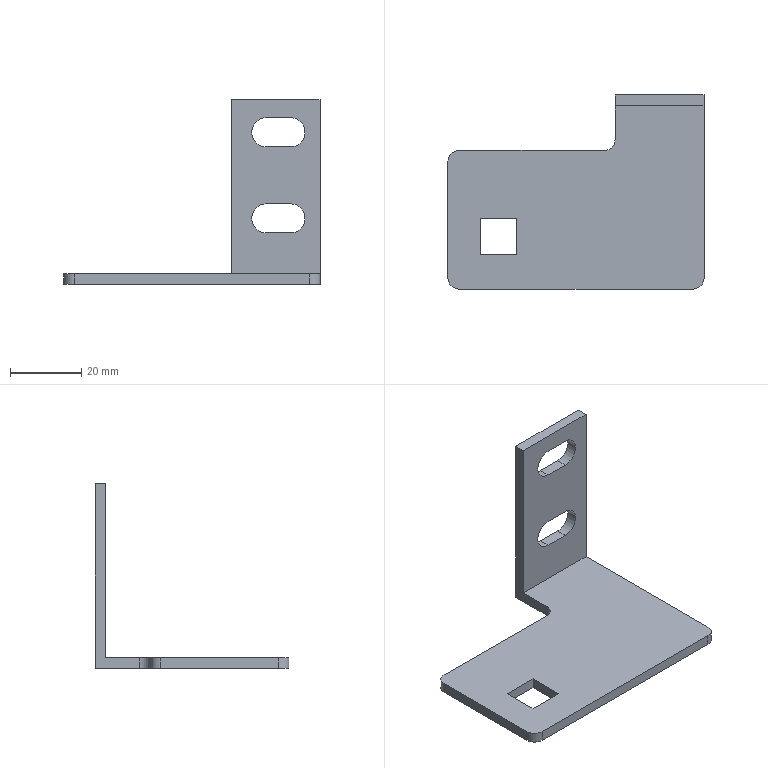Component | SolidWorks | MotorHeadBracket-1 | 1 solid | 26 faces | box 72 x 54.5 x 52 mm | volume 12286 mm3 | plane 18 | cylinder 8 | commonest cylinder face diameters 6 x4 8.2 x4
build123d program:
from build123d import *

# Parameters (mm, degrees)
SKETCH2_W           = 10.2
SKETCH2_H           = 10.2
BOSS_EXTRUDE1_DEPTH = 3
FILLET1_R           = 3
SKETCH3_W           = 25
SKETCH3_H           = 3
BOSS_EXTRUDE2_DEPTH = 52
CUT_EXTRUDE1_DEPTH  = 12


with BuildPart() as part:
    # Sketch2 → Boss-Extrude1 (new body)
    with BuildSketch(Plane.XY):
        Polygon((0, 0), (0, 39), (47, 39), (47, 54.5), (72, 54.5), (72, 0), align=None)
        with Locations((14.2, 14.8)):
            Rectangle(SKETCH2_W, SKETCH2_H, mode=Mode.SUBTRACT)
    extrude(amount=BOSS_EXTRUDE1_DEPTH)

    # Fillet1
    fillet1_edges = [part.edges().sort_by_distance(p)[0] for p in [
        (0, 0, 1.5),
        (0, 39, 1.5),
        (47, 39, 1.5),
        (72, 0, 1.5),
    ]]
    fillet(fillet1_edges, radius=FILLET1_R)

    # Sketch3 → Boss-Extrude2 (add)
    with BuildSketch(Plane.XY):
        with Locations((59.5, 53)):
            Rectangle(SKETCH3_W, SKETCH3_H)
    extrude(amount=BOSS_EXTRUDE2_DEPTH)

    # Sketch4 → Cut-Extrude1 (cut)
    with BuildSketch(Plane(origin=(0, 54.5, 0), x_dir=(1, 0, 0), z_dir=(0, 1, 0))):
        with BuildLine():
            Line((63.7, -46.9), (56.9, -46.9))
            ThreePointArc((56.9, -46.9), (52.8, -42.8), (56.9, -38.7))
            Line((56.9, -38.7), (63.7, -38.7))
            ThreePointArc((63.7, -38.7), (67.8, -42.8), (63.7, -46.9))
        make_face()
        with BuildLine():
            Line((63.7, -22.7), (56.9, -22.7))
            ThreePointArc((56.9, -22.7), (52.8, -18.6), (56.9, -14.5))
            Line((56.9, -14.5), (63.7, -14.5))
            ThreePointArc((63.7, -14.5), (67.8, -18.6), (63.7, -22.7))
        make_face()
    extrude(amount=-CUT_EXTRUDE1_DEPTH, mode=Mode.SUBTRACT)


solid = part.part

# Placed as in the assembly
solid = solid.moved(Location((-79.293, -47.753, 1574.064), (0, 0, 0)))
STEP:
#1=COLOUR_RGB('',0.7922,0.8196,0.9333);
#2=FILL_AREA_STYLE_COLOUR('',#1);
#3=FILL_AREA_STYLE('',(#2));
#4=SURFACE_STYLE_FILL_AREA(#3);
#5=SURFACE_SIDE_STYLE('',(#4));
#6=SURFACE_STYLE_USAGE(.BOTH.,#5);
#7=PRESENTATION_STYLE_ASSIGNMENT((#6));
#8=CARTESIAN_POINT('',(-2.362,-1.498,62.089));
#9=VERTEX_POINT('',#8);
#10=CARTESIAN_POINT('',(-2.362,-1.097,62.089));
#11=VERTEX_POINT('',#10);
#12=CARTESIAN_POINT('',(-2.362,-1.097,62.089));
#13=DIRECTION('',(0.,1.,0.));
#14=VECTOR('',#13,39.37);
#15=LINE('',#12,#14);
#16=EDGE_CURVE('',#9,#11,#15,.T.);
#17=ORIENTED_EDGE('',*,*,#16,.F.);
#18=CARTESIAN_POINT('',(-2.764,-1.498,62.089));
#19=VERTEX_POINT('',#18);
#20=CARTESIAN_POINT('',(-2.764,-1.498,62.089));
#21=DIRECTION('',(1.,0.,0.));
#22=VECTOR('',#21,39.37);
#23=LINE('',#20,#22);
#24=EDGE_CURVE('',#19,#9,#23,.T.);
#25=ORIENTED_EDGE('',*,*,#24,.F.);
#26=CARTESIAN_POINT('',(-2.764,-1.097,62.089));
#27=VERTEX_POINT('',#26);
#28=CARTESIAN_POINT('',(-2.764,-1.097,62.089));
#29=DIRECTION('',(0.,-1.,0.));
#30=VECTOR('',#29,39.37);
#31=LINE('',#28,#30);
#32=EDGE_CURVE('',#27,#19,#31,.T.);
#33=ORIENTED_EDGE('',*,*,#32,.F.);
#34=CARTESIAN_POINT('',(-2.764,-1.097,62.089));
#35=DIRECTION('',(-1.,-0.,0.));
#36=VECTOR('',#35,39.37);
#37=LINE('',#34,#36);
#38=EDGE_CURVE('',#11,#27,#37,.T.);
#39=ORIENTED_EDGE('',*,*,#38,.F.);
#40=EDGE_LOOP('',(#17,#25,#33,#39));
#41=FACE_BOUND('',#40,.T.);
#42=CARTESIAN_POINT('',(-1.271,0.1475,62.089));
#43=VERTEX_POINT('',#42);
#44=CARTESIAN_POINT('',(-0.2871,0.1475,62.089));
#45=VERTEX_POINT('',#44);
#46=CARTESIAN_POINT('',(-3.122,0.1475,62.089));
#47=DIRECTION('',(1.,0.,0.));
#48=VECTOR('',#47,39.37);
#49=LINE('',#46,#48);
#50=EDGE_CURVE('',#43,#45,#49,.T.);
#51=ORIENTED_EDGE('',*,*,#50,.F.);
#52=CARTESIAN_POINT('',(-1.271,-0.2265,62.089));
#53=VERTEX_POINT('',#52);
#54=CARTESIAN_POINT('',(-1.271,0.2656,62.089));
#55=DIRECTION('',(0.,-1.,0.));
#56=VECTOR('',#55,39.37);
#57=LINE('',#54,#56);
#58=EDGE_CURVE('',#43,#53,#57,.T.);
#59=ORIENTED_EDGE('',*,*,#58,.T.);
#60=CARTESIAN_POINT('',(-1.39,-0.3446,62.089));
#61=VERTEX_POINT('',#60);
#62=CARTESIAN_POINT('',(-1.39,-0.2265,62.089));
#63=DIRECTION('',(0.,0.,-1.));
#64=DIRECTION('',(-1.,0.,0.));
#65=AXIS2_PLACEMENT_3D('',#62,#63,#64);
#66=CIRCLE('',#65,0.1181);
#67=EDGE_CURVE('',#53,#61,#66,.T.);
#68=ORIENTED_EDGE('',*,*,#67,.T.);
#69=CARTESIAN_POINT('',(-3.004,-0.3446,62.089));
#70=VERTEX_POINT('',#69);
#71=CARTESIAN_POINT('',(-3.122,-0.3446,62.089));
#72=DIRECTION('',(-1.,0.,0.));
#73=VECTOR('',#72,39.37);
#74=LINE('',#71,#73);
#75=EDGE_CURVE('',#61,#70,#74,.T.);
#76=ORIENTED_EDGE('',*,*,#75,.T.);
#77=CARTESIAN_POINT('',(-3.122,-0.4627,62.089));
#78=VERTEX_POINT('',#77);
#79=CARTESIAN_POINT('',(-3.004,-0.4627,62.089));
#80=DIRECTION('',(0.,0.,1.));
#81=DIRECTION('',(-1.,0.,0.));
#82=AXIS2_PLACEMENT_3D('',#79,#80,#81);
#83=CIRCLE('',#82,0.1181);
#84=EDGE_CURVE('',#70,#78,#83,.T.);
#85=ORIENTED_EDGE('',*,*,#84,.T.);
#86=CARTESIAN_POINT('',(-3.122,-1.762,62.089));
#87=VERTEX_POINT('',#86);
#88=CARTESIAN_POINT('',(-3.122,-1.88,62.089));
#89=DIRECTION('',(0.,-1.,0.));
#90=VECTOR('',#89,39.37);
#91=LINE('',#88,#90);
#92=EDGE_CURVE('',#78,#87,#91,.T.);
#93=ORIENTED_EDGE('',*,*,#92,.T.);
#94=CARTESIAN_POINT('',(-3.004,-1.88,62.089));
#95=VERTEX_POINT('',#94);
#96=CARTESIAN_POINT('',(-3.004,-1.762,62.089));
#97=DIRECTION('',(0.,0.,1.));
#98=DIRECTION('',(-1.,0.,0.));
#99=AXIS2_PLACEMENT_3D('',#96,#97,#98);
#100=CIRCLE('',#99,0.1181);
#101=EDGE_CURVE('',#87,#95,#100,.T.);
#102=ORIENTED_EDGE('',*,*,#101,.T.);
#103=CARTESIAN_POINT('',(-0.4053,-1.88,62.089));
#104=VERTEX_POINT('',#103);
#105=CARTESIAN_POINT('',(-0.2871,-1.88,62.089));
#106=DIRECTION('',(1.,0.,0.));
#107=VECTOR('',#106,39.37);
#108=LINE('',#105,#107);
#109=EDGE_CURVE('',#95,#104,#108,.T.);
#110=ORIENTED_EDGE('',*,*,#109,.T.);
#111=CARTESIAN_POINT('',(-0.2871,-1.762,62.089));
#112=VERTEX_POINT('',#111);
#113=CARTESIAN_POINT('',(-0.4053,-1.762,62.089));
#114=DIRECTION('',(0.,0.,1.));
#115=DIRECTION('',(-1.,0.,0.));
#116=AXIS2_PLACEMENT_3D('',#113,#114,#115);
#117=CIRCLE('',#116,0.1181);
#118=EDGE_CURVE('',#104,#112,#117,.T.);
#119=ORIENTED_EDGE('',*,*,#118,.T.);
#120=CARTESIAN_POINT('',(-0.2871,-1.88,62.089));
#121=DIRECTION('',(-0.,1.,0.));
#122=VECTOR('',#121,39.37);
#123=LINE('',#120,#122);
#124=EDGE_CURVE('',#112,#45,#123,.T.);
#125=ORIENTED_EDGE('',*,*,#124,.T.);
#126=EDGE_LOOP('',(#51,#59,#68,#76,#85,#93,#102,#110,#119,#125));
#127=FACE_OUTER_BOUND('',#126,.T.);
#128=CARTESIAN_POINT('',(-3.122,-1.88,62.089));
#129=DIRECTION('',(0.,0.,-1.));
#130=DIRECTION('',(-1.,0.,0.));
#131=AXIS2_PLACEMENT_3D('',#128,#129,#130);
#132=PLANE('',#131);
#133=ADVANCED_FACE('',(#41,#127),#132,.F.);
#134=CARTESIAN_POINT('',(-0.2871,0.2656,61.971));
#135=VERTEX_POINT('',#134);
#136=CARTESIAN_POINT('',(-1.271,0.2656,61.971));
#137=VERTEX_POINT('',#136);
#138=CARTESIAN_POINT('',(-0.2871,0.2656,61.971));
#139=DIRECTION('',(-1.,0.,0.));
#140=VECTOR('',#139,39.37);
#141=LINE('',#138,#140);
#142=EDGE_CURVE('',#135,#137,#141,.T.);
#143=ORIENTED_EDGE('',*,*,#142,.F.);
#144=CARTESIAN_POINT('',(-0.2871,-1.762,61.971));
#145=VERTEX_POINT('',#144);
#146=CARTESIAN_POINT('',(-0.2871,-1.88,61.971));
#147=DIRECTION('',(-0.,1.,0.));
#148=VECTOR('',#147,39.37);
#149=LINE('',#146,#148);
#150=EDGE_CURVE('',#145,#135,#149,.T.);
#151=ORIENTED_EDGE('',*,*,#150,.F.);
#152=CARTESIAN_POINT('',(-0.4053,-1.88,61.971));
#153=VERTEX_POINT('',#152);
#154=CARTESIAN_POINT('',(-0.4053,-1.762,61.971));
#155=DIRECTION('',(0.,0.,-1.));
#156=DIRECTION('',(-1.,0.,0.));
#157=AXIS2_PLACEMENT_3D('',#154,#155,#156);
#158=CIRCLE('',#157,0.1181);
#159=EDGE_CURVE('',#145,#153,#158,.T.);
#160=ORIENTED_EDGE('',*,*,#159,.T.);
#161=CARTESIAN_POINT('',(-3.004,-1.88,61.971));
#162=VERTEX_POINT('',#161);
#163=CARTESIAN_POINT('',(-0.2871,-1.88,61.971));
#164=DIRECTION('',(1.,0.,0.));
#165=VECTOR('',#164,39.37);
#166=LINE('',#163,#165);
#167=EDGE_CURVE('',#162,#153,#166,.T.);
#168=ORIENTED_EDGE('',*,*,#167,.F.);
#169=CARTESIAN_POINT('',(-3.122,-1.762,61.971));
#170=VERTEX_POINT('',#169);
#171=CARTESIAN_POINT('',(-3.004,-1.762,61.971));
#172=DIRECTION('',(0.,0.,-1.));
#173=DIRECTION('',(-1.,0.,0.));
#174=AXIS2_PLACEMENT_3D('',#171,#172,#173);
#175=CIRCLE('',#174,0.1181);
#176=EDGE_CURVE('',#162,#170,#175,.T.);
#177=ORIENTED_EDGE('',*,*,#176,.T.);
#178=CARTESIAN_POINT('',(-3.122,-0.4627,61.971));
#179=VERTEX_POINT('',#178);
#180=CARTESIAN_POINT('',(-3.122,-1.88,61.971));
#181=DIRECTION('',(0.,-1.,0.));
#182=VECTOR('',#181,39.37);
#183=LINE('',#180,#182);
#184=EDGE_CURVE('',#179,#170,#183,.T.);
#185=ORIENTED_EDGE('',*,*,#184,.F.);
#186=CARTESIAN_POINT('',(-3.004,-0.3446,61.971));
#187=VERTEX_POINT('',#186);
#188=CARTESIAN_POINT('',(-3.004,-0.4627,61.971));
#189=DIRECTION('',(0.,0.,-1.));
#190=DIRECTION('',(-1.,0.,0.));
#191=AXIS2_PLACEMENT_3D('',#188,#189,#190);
#192=CIRCLE('',#191,0.1181);
#193=EDGE_CURVE('',#179,#187,#192,.T.);
#194=ORIENTED_EDGE('',*,*,#193,.T.);
#195=CARTESIAN_POINT('',(-1.39,-0.3446,61.971));
#196=VERTEX_POINT('',#195);
#197=CARTESIAN_POINT('',(-3.122,-0.3446,61.971));
#198=DIRECTION('',(-1.,0.,0.));
#199=VECTOR('',#198,39.37);
#200=LINE('',#197,#199);
#201=EDGE_CURVE('',#196,#187,#200,.T.);
#202=ORIENTED_EDGE('',*,*,#201,.F.);
#203=CARTESIAN_POINT('',(-1.271,-0.2265,61.971));
#204=VERTEX_POINT('',#203);
#205=CARTESIAN_POINT('',(-1.39,-0.2265,61.971));
#206=DIRECTION('',(0.,0.,1.));
#207=DIRECTION('',(-1.,0.,0.));
#208=AXIS2_PLACEMENT_3D('',#205,#206,#207);
#209=CIRCLE('',#208,0.1181);
#210=EDGE_CURVE('',#196,#204,#209,.T.);
#211=ORIENTED_EDGE('',*,*,#210,.T.);
#212=CARTESIAN_POINT('',(-1.271,0.2656,61.971));
#213=DIRECTION('',(0.,-1.,0.));
#214=VECTOR('',#213,39.37);
#215=LINE('',#212,#214);
#216=EDGE_CURVE('',#137,#204,#215,.T.);
#217=ORIENTED_EDGE('',*,*,#216,.F.);
#218=EDGE_LOOP('',(#143,#151,#160,#168,#177,#185,#194,#202,#211,#217));
#219=FACE_OUTER_BOUND('',#218,.T.);
#220=CARTESIAN_POINT('',(-2.764,-1.498,61.971));
#221=VERTEX_POINT('',#220);
#222=CARTESIAN_POINT('',(-2.362,-1.498,61.971));
#223=VERTEX_POINT('',#222);
#224=CARTESIAN_POINT('',(-2.764,-1.498,61.971));
#225=DIRECTION('',(1.,0.,0.));
#226=VECTOR('',#225,39.37);
#227=LINE('',#224,#226);
#228=EDGE_CURVE('',#221,#223,#227,.T.);
#229=ORIENTED_EDGE('',*,*,#228,.T.);
#230=CARTESIAN_POINT('',(-2.362,-1.097,61.971));
#231=VERTEX_POINT('',#230);
#232=CARTESIAN_POINT('',(-2.362,-1.097,61.971));
#233=DIRECTION('',(0.,1.,0.));
#234=VECTOR('',#233,39.37);
#235=LINE('',#232,#234);
#236=EDGE_CURVE('',#223,#231,#235,.T.);
#237=ORIENTED_EDGE('',*,*,#236,.T.);
#238=CARTESIAN_POINT('',(-2.764,-1.097,61.971));
#239=VERTEX_POINT('',#238);
#240=CARTESIAN_POINT('',(-2.764,-1.097,61.971));
#241=DIRECTION('',(-1.,-0.,0.));
#242=VECTOR('',#241,39.37);
#243=LINE('',#240,#242);
#244=EDGE_CURVE('',#231,#239,#243,.T.);
#245=ORIENTED_EDGE('',*,*,#244,.T.);
#246=CARTESIAN_POINT('',(-2.764,-1.097,61.971));
#247=DIRECTION('',(0.,-1.,0.));
#248=VECTOR('',#247,39.37);
#249=LINE('',#246,#248);
#250=EDGE_CURVE('',#239,#221,#249,.T.);
#251=ORIENTED_EDGE('',*,*,#250,.T.);
#252=EDGE_LOOP('',(#229,#237,#245,#251));
#253=FACE_BOUND('',#252,.T.);
#254=CARTESIAN_POINT('',(-3.122,-1.88,61.971));
#255=DIRECTION('',(0.,0.,-1.));
#256=DIRECTION('',(-1.,0.,0.));
#257=AXIS2_PLACEMENT_3D('',#254,#255,#256);
#258=PLANE('',#257);
#259=ADVANCED_FACE('',(#219,#253),#258,.T.);
#260=ORIENTED_EDGE('',*,*,#167,.T.);
#261=CARTESIAN_POINT('',(-0.4053,-1.88,62.089));
#262=DIRECTION('',(0.,0.,1.));
#263=VECTOR('',#262,39.37);
#264=LINE('',#261,#263);
#265=EDGE_CURVE('',#153,#104,#264,.T.);
#266=ORIENTED_EDGE('',*,*,#265,.T.);
#267=ORIENTED_EDGE('',*,*,#109,.F.);
#268=CARTESIAN_POINT('',(-3.004,-1.88,62.089));
#269=DIRECTION('',(0.,0.,-1.));
#270=VECTOR('',#269,39.37);
#271=LINE('',#268,#270);
#272=EDGE_CURVE('',#95,#162,#271,.T.);
#273=ORIENTED_EDGE('',*,*,#272,.T.);
#274=EDGE_LOOP('',(#260,#266,#267,#273));
#275=FACE_OUTER_BOUND('',#274,.T.);
#276=CARTESIAN_POINT('',(-0.2871,-1.88,62.089));
#277=DIRECTION('',(-0.,1.,0.));
#278=DIRECTION('',(-1.,-0.,0.));
#279=AXIS2_PLACEMENT_3D('',#276,#277,#278);
#280=PLANE('',#279);
#281=ADVANCED_FACE('',(#275),#280,.F.);
#282=CARTESIAN_POINT('',(-0.2871,0.2656,64.018));
#283=VERTEX_POINT('',#282);
#284=CARTESIAN_POINT('',(-0.2871,0.2656,62.089));
#285=DIRECTION('',(0.,0.,-1.));
#286=VECTOR('',#285,39.37);
#287=LINE('',#284,#286);
#288=EDGE_CURVE('',#283,#135,#287,.T.);
#289=ORIENTED_EDGE('',*,*,#288,.F.);
#290=CARTESIAN_POINT('',(-0.2871,0.1475,64.018));
#291=VERTEX_POINT('',#290);
#292=CARTESIAN_POINT('',(-0.2871,0.1475,64.018));
#293=DIRECTION('',(-0.,1.,0.));
#294=VECTOR('',#293,39.37);
#295=LINE('',#292,#294);
#296=EDGE_CURVE('',#291,#283,#295,.T.);
#297=ORIENTED_EDGE('',*,*,#296,.F.);
#298=CARTESIAN_POINT('',(-0.2871,0.1475,64.018));
#299=DIRECTION('',(0.,0.,-1.));
#300=VECTOR('',#299,39.37);
#301=LINE('',#298,#300);
#302=EDGE_CURVE('',#291,#45,#301,.T.);
#303=ORIENTED_EDGE('',*,*,#302,.T.);
#304=ORIENTED_EDGE('',*,*,#124,.F.);
#305=CARTESIAN_POINT('',(-0.2871,-1.762,62.089));
#306=DIRECTION('',(0.,0.,-1.));
#307=VECTOR('',#306,39.37);
#308=LINE('',#305,#307);
#309=EDGE_CURVE('',#112,#145,#308,.T.);
#310=ORIENTED_EDGE('',*,*,#309,.T.);
#311=ORIENTED_EDGE('',*,*,#150,.T.);
#312=EDGE_LOOP('',(#289,#297,#303,#304,#310,#311));
#313=FACE_OUTER_BOUND('',#312,.T.);
#314=CARTESIAN_POINT('',(-0.2871,-1.88,62.089));
#315=DIRECTION('',(-1.,-0.,0.));
#316=DIRECTION('',(0.,-1.,0.));
#317=AXIS2_PLACEMENT_3D('',#314,#315,#316);
#318=PLANE('',#317);
#319=ADVANCED_FACE('',(#313),#318,.F.);
#320=CARTESIAN_POINT('',(-0.6139,0.2656,63.495));
#321=VERTEX_POINT('',#320);
#322=CARTESIAN_POINT('',(-0.8816,0.2656,63.495));
#323=VERTEX_POINT('',#322);
#324=CARTESIAN_POINT('',(-0.6139,0.2656,63.495));
#325=DIRECTION('',(-1.,0.,0.));
#326=VECTOR('',#325,39.37);
#327=LINE('',#324,#326);
#328=EDGE_CURVE('',#321,#323,#327,.T.);
#329=ORIENTED_EDGE('',*,*,#328,.F.);
#330=CARTESIAN_POINT('',(-0.6139,0.2656,63.817));
#331=VERTEX_POINT('',#330);
#332=CARTESIAN_POINT('',(-0.6139,0.2656,63.656));
#333=DIRECTION('',(0.,1.,0.));
#334=DIRECTION('',(0.,0.,1.));
#335=AXIS2_PLACEMENT_3D('',#332,#333,#334);
#336=CIRCLE('',#335,0.1614);
#337=EDGE_CURVE('',#331,#321,#336,.T.);
#338=ORIENTED_EDGE('',*,*,#337,.F.);
#339=CARTESIAN_POINT('',(-0.8816,0.2656,63.817));
#340=VERTEX_POINT('',#339);
#341=CARTESIAN_POINT('',(-0.6139,0.2656,63.817));
#342=DIRECTION('',(1.,0.,0.));
#343=VECTOR('',#342,39.37);
#344=LINE('',#341,#343);
#345=EDGE_CURVE('',#340,#331,#344,.T.);
#346=ORIENTED_EDGE('',*,*,#345,.F.);
#347=CARTESIAN_POINT('',(-0.8816,0.2656,63.656));
#348=DIRECTION('',(0.,1.,0.));
#349=DIRECTION('',(0.,0.,1.));
#350=AXIS2_PLACEMENT_3D('',#347,#348,#349);
#351=CIRCLE('',#350,0.1614);
#352=EDGE_CURVE('',#323,#340,#351,.T.);
#353=ORIENTED_EDGE('',*,*,#352,.F.);
#354=EDGE_LOOP('',(#329,#338,#346,#353));
#355=FACE_BOUND('',#354,.T.);
#356=CARTESIAN_POINT('',(-0.6139,0.2656,62.542));
#357=VERTEX_POINT('',#356);
#358=CARTESIAN_POINT('',(-0.8816,0.2656,62.542));
#359=VERTEX_POINT('',#358);
#360=CARTESIAN_POINT('',(-0.6139,0.2656,62.542));
#361=DIRECTION('',(-1.,0.,0.));
#362=VECTOR('',#361,39.37);
#363=LINE('',#360,#362);
#364=EDGE_CURVE('',#357,#359,#363,.T.);
#365=ORIENTED_EDGE('',*,*,#364,.F.);
#366=CARTESIAN_POINT('',(-0.6139,0.2656,62.865));
#367=VERTEX_POINT('',#366);
#368=CARTESIAN_POINT('',(-0.6139,0.2656,62.703));
#369=DIRECTION('',(0.,1.,0.));
#370=DIRECTION('',(0.,0.,1.));
#371=AXIS2_PLACEMENT_3D('',#368,#369,#370);
#372=CIRCLE('',#371,0.1614);
#373=EDGE_CURVE('',#367,#357,#372,.T.);
#374=ORIENTED_EDGE('',*,*,#373,.F.);
#375=CARTESIAN_POINT('',(-0.8816,0.2656,62.865));
#376=VERTEX_POINT('',#375);
#377=CARTESIAN_POINT('',(-0.6139,0.2656,62.865));
#378=DIRECTION('',(1.,0.,0.));
#379=VECTOR('',#378,39.37);
#380=LINE('',#377,#379);
#381=EDGE_CURVE('',#376,#367,#380,.T.);
#382=ORIENTED_EDGE('',*,*,#381,.F.);
#383=CARTESIAN_POINT('',(-0.8816,0.2656,62.703));
#384=DIRECTION('',(0.,1.,0.));
#385=DIRECTION('',(0.,0.,1.));
#386=AXIS2_PLACEMENT_3D('',#383,#384,#385);
#387=CIRCLE('',#386,0.1614);
#388=EDGE_CURVE('',#359,#376,#387,.T.);
#389=ORIENTED_EDGE('',*,*,#388,.F.);
#390=EDGE_LOOP('',(#365,#374,#382,#389));
#391=FACE_BOUND('',#390,.T.);
#392=ORIENTED_EDGE('',*,*,#142,.T.);
#393=CARTESIAN_POINT('',(-1.271,0.2656,64.018));
#394=VERTEX_POINT('',#393);
#395=CARTESIAN_POINT('',(-1.271,0.2656,62.089));
#396=DIRECTION('',(0.,0.,-1.));
#397=VECTOR('',#396,39.37);
#398=LINE('',#395,#397);
#399=EDGE_CURVE('',#394,#137,#398,.T.);
#400=ORIENTED_EDGE('',*,*,#399,.F.);
#401=CARTESIAN_POINT('',(-0.2871,0.2656,64.018));
#402=DIRECTION('',(-1.,0.,0.));
#403=VECTOR('',#402,39.37);
#404=LINE('',#401,#403);
#405=EDGE_CURVE('',#283,#394,#404,.T.);
#406=ORIENTED_EDGE('',*,*,#405,.F.);
#407=ORIENTED_EDGE('',*,*,#288,.T.);
#408=EDGE_LOOP('',(#392,#400,#406,#407));
#409=FACE_OUTER_BOUND('',#408,.T.);
#410=CARTESIAN_POINT('',(-0.2871,0.2656,62.089));
#411=DIRECTION('',(0.,-1.,0.));
#412=DIRECTION('',(0.,0.,-1.));
#413=AXIS2_PLACEMENT_3D('',#410,#411,#412);
#414=PLANE('',#413);
#415=ADVANCED_FACE('',(#355,#391,#409),#414,.F.);
#416=ORIENTED_EDGE('',*,*,#216,.T.);
#417=CARTESIAN_POINT('',(-1.271,-0.2265,62.089));
#418=DIRECTION('',(0.,0.,1.));
#419=VECTOR('',#418,39.37);
#420=LINE('',#417,#419);
#421=EDGE_CURVE('',#204,#53,#420,.T.);
#422=ORIENTED_EDGE('',*,*,#421,.T.);
#423=ORIENTED_EDGE('',*,*,#58,.F.);
#424=CARTESIAN_POINT('',(-1.271,0.1475,64.018));
#425=VERTEX_POINT('',#424);
#426=CARTESIAN_POINT('',(-1.271,0.1475,64.018));
#427=DIRECTION('',(0.,0.,-1.));
#428=VECTOR('',#427,39.37);
#429=LINE('',#426,#428);
#430=EDGE_CURVE('',#425,#43,#429,.T.);
#431=ORIENTED_EDGE('',*,*,#430,.F.);
#432=CARTESIAN_POINT('',(-1.271,0.2656,64.018));
#433=DIRECTION('',(0.,-1.,0.));
#434=VECTOR('',#433,39.37);
#435=LINE('',#432,#434);
#436=EDGE_CURVE('',#394,#425,#435,.T.);
#437=ORIENTED_EDGE('',*,*,#436,.F.);
#438=ORIENTED_EDGE('',*,*,#399,.T.);
#439=EDGE_LOOP('',(#416,#422,#423,#431,#437,#438));
#440=FACE_OUTER_BOUND('',#439,.T.);
#441=CARTESIAN_POINT('',(-1.271,0.2656,62.089));
#442=DIRECTION('',(1.,0.,0.));
#443=DIRECTION('',(0.,0.,-1.));
#444=AXIS2_PLACEMENT_3D('',#441,#442,#443);
#445=PLANE('',#444);
#446=ADVANCED_FACE('',(#440),#445,.F.);
#447=ORIENTED_EDGE('',*,*,#201,.T.);
#448=CARTESIAN_POINT('',(-3.004,-0.3446,62.089));
#449=DIRECTION('',(0.,0.,1.));
#450=VECTOR('',#449,39.37);
#451=LINE('',#448,#450);
#452=EDGE_CURVE('',#187,#70,#451,.T.);
#453=ORIENTED_EDGE('',*,*,#452,.T.);
#454=ORIENTED_EDGE('',*,*,#75,.F.);
#455=CARTESIAN_POINT('',(-1.39,-0.3446,61.971));
#456=DIRECTION('',(0.,0.,-1.));
#457=VECTOR('',#456,39.37);
#458=LINE('',#455,#457);
#459=EDGE_CURVE('',#61,#196,#458,.T.);
#460=ORIENTED_EDGE('',*,*,#459,.T.);
#461=EDGE_LOOP('',(#447,#453,#454,#460));
#462=FACE_OUTER_BOUND('',#461,.T.);
#463=CARTESIAN_POINT('',(-3.122,-0.3446,62.089));
#464=DIRECTION('',(0.,-1.,0.));
#465=DIRECTION('',(0.,0.,-1.));
#466=AXIS2_PLACEMENT_3D('',#463,#464,#465);
#467=PLANE('',#466);
#468=ADVANCED_FACE('',(#462),#467,.F.);
#469=ORIENTED_EDGE('',*,*,#184,.T.);
#470=CARTESIAN_POINT('',(-3.122,-1.762,62.089));
#471=DIRECTION('',(0.,0.,1.));
#472=VECTOR('',#471,39.37);
#473=LINE('',#470,#472);
#474=EDGE_CURVE('',#170,#87,#473,.T.);
#475=ORIENTED_EDGE('',*,*,#474,.T.);
#476=ORIENTED_EDGE('',*,*,#92,.F.);
#477=CARTESIAN_POINT('',(-3.122,-0.4627,62.089));
#478=DIRECTION('',(0.,0.,-1.));
#479=VECTOR('',#478,39.37);
#480=LINE('',#477,#479);
#481=EDGE_CURVE('',#78,#179,#480,.T.);
#482=ORIENTED_EDGE('',*,*,#481,.T.);
#483=EDGE_LOOP('',(#469,#475,#476,#482));
#484=FACE_OUTER_BOUND('',#483,.T.);
#485=CARTESIAN_POINT('',(-3.122,-1.88,62.089));
#486=DIRECTION('',(1.,0.,0.));
#487=DIRECTION('',(0.,0.,-1.));
#488=AXIS2_PLACEMENT_3D('',#485,#486,#487);
#489=PLANE('',#488);
#490=ADVANCED_FACE('',(#484),#489,.F.);
#491=ORIENTED_EDGE('',*,*,#236,.F.);
#492=CARTESIAN_POINT('',(-2.362,-1.498,62.089));
#493=DIRECTION('',(0.,0.,-1.));
#494=VECTOR('',#493,39.37);
#495=LINE('',#492,#494);
#496=EDGE_CURVE('',#9,#223,#495,.T.);
#497=ORIENTED_EDGE('',*,*,#496,.F.);
#498=ORIENTED_EDGE('',*,*,#16,.T.);
#499=CARTESIAN_POINT('',(-2.362,-1.097,62.089));
#500=DIRECTION('',(0.,0.,-1.));
#501=VECTOR('',#500,39.37);
#502=LINE('',#499,#501);
#503=EDGE_CURVE('',#11,#231,#502,.T.);
#504=ORIENTED_EDGE('',*,*,#503,.T.);
#505=EDGE_LOOP('',(#491,#497,#498,#504));
#506=FACE_OUTER_BOUND('',#505,.T.);
#507=CARTESIAN_POINT('',(-2.362,-1.097,62.089));
#508=DIRECTION('',(-1.,0.,0.));
#509=DIRECTION('',(0.,0.,1.));
#510=AXIS2_PLACEMENT_3D('',#507,#508,#509);
#511=PLANE('',#510);
#512=ADVANCED_FACE('',(#506),#511,.T.);
#513=ORIENTED_EDGE('',*,*,#244,.F.);
#514=ORIENTED_EDGE('',*,*,#503,.F.);
#515=ORIENTED_EDGE('',*,*,#38,.T.);
#516=CARTESIAN_POINT('',(-2.764,-1.097,62.089));
#517=DIRECTION('',(0.,0.,-1.));
#518=VECTOR('',#517,39.37);
#519=LINE('',#516,#518);
#520=EDGE_CURVE('',#27,#239,#519,.T.);
#521=ORIENTED_EDGE('',*,*,#520,.T.);
#522=EDGE_LOOP('',(#513,#514,#515,#521));
#523=FACE_OUTER_BOUND('',#522,.T.);
#524=CARTESIAN_POINT('',(-2.764,-1.097,62.089));
#525=DIRECTION('',(0.,-1.,0.));
#526=DIRECTION('',(1.,0.,0.));
#527=AXIS2_PLACEMENT_3D('',#524,#525,#526);
#528=PLANE('',#527);
#529=ADVANCED_FACE('',(#523),#528,.T.);
#530=ORIENTED_EDGE('',*,*,#250,.F.);
#531=ORIENTED_EDGE('',*,*,#520,.F.);
#532=ORIENTED_EDGE('',*,*,#32,.T.);
#533=CARTESIAN_POINT('',(-2.764,-1.498,62.089));
#534=DIRECTION('',(0.,0.,-1.));
#535=VECTOR('',#534,39.37);
#536=LINE('',#533,#535);
#537=EDGE_CURVE('',#19,#221,#536,.T.);
#538=ORIENTED_EDGE('',*,*,#537,.T.);
#539=EDGE_LOOP('',(#530,#531,#532,#538));
#540=FACE_OUTER_BOUND('',#539,.T.);
#541=CARTESIAN_POINT('',(-2.764,-1.097,62.089));
#542=DIRECTION('',(1.,0.,0.));
#543=DIRECTION('',(-0.,1.,0.));
#544=AXIS2_PLACEMENT_3D('',#541,#542,#543);
#545=PLANE('',#544);
#546=ADVANCED_FACE('',(#540),#545,.T.);
#547=ORIENTED_EDGE('',*,*,#228,.F.);
#548=ORIENTED_EDGE('',*,*,#537,.F.);
#549=ORIENTED_EDGE('',*,*,#24,.T.);
#550=ORIENTED_EDGE('',*,*,#496,.T.);
#551=EDGE_LOOP('',(#547,#548,#549,#550));
#552=FACE_OUTER_BOUND('',#551,.T.);
#553=CARTESIAN_POINT('',(-2.764,-1.498,62.089));
#554=DIRECTION('',(0.,1.,0.));
#555=DIRECTION('',(0.,0.,1.));
#556=AXIS2_PLACEMENT_3D('',#553,#554,#555);
#557=PLANE('',#556);
#558=ADVANCED_FACE('',(#552),#557,.T.);
#559=ORIENTED_EDGE('',*,*,#118,.F.);
#560=ORIENTED_EDGE('',*,*,#265,.F.);
#561=ORIENTED_EDGE('',*,*,#159,.F.);
#562=ORIENTED_EDGE('',*,*,#309,.F.);
#563=EDGE_LOOP('',(#559,#560,#561,#562));
#564=FACE_OUTER_BOUND('',#563,.T.);
#565=CARTESIAN_POINT('',(-0.4053,-1.762,62.089));
#566=DIRECTION('',(0.,0.,-1.));
#567=DIRECTION('',(-1.,0.,0.));
#568=AXIS2_PLACEMENT_3D('',#565,#566,#567);
#569=CYLINDRICAL_SURFACE('',#568,0.1181);
#570=ADVANCED_FACE('',(#564),#569,.T.);
#571=ORIENTED_EDGE('',*,*,#101,.F.);
#572=ORIENTED_EDGE('',*,*,#474,.F.);
#573=ORIENTED_EDGE('',*,*,#176,.F.);
#574=ORIENTED_EDGE('',*,*,#272,.F.);
#575=EDGE_LOOP('',(#571,#572,#573,#574));
#576=FACE_OUTER_BOUND('',#575,.T.);
#577=CARTESIAN_POINT('',(-3.004,-1.762,62.089));
#578=DIRECTION('',(0.,0.,-1.));
#579=DIRECTION('',(-1.,0.,0.));
#580=AXIS2_PLACEMENT_3D('',#577,#578,#579);
#581=CYLINDRICAL_SURFACE('',#580,0.1181);
#582=ADVANCED_FACE('',(#576),#581,.T.);
#583=ORIENTED_EDGE('',*,*,#84,.F.);
#584=ORIENTED_EDGE('',*,*,#452,.F.);
#585=ORIENTED_EDGE('',*,*,#193,.F.);
#586=ORIENTED_EDGE('',*,*,#481,.F.);
#587=EDGE_LOOP('',(#583,#584,#585,#586));
#588=FACE_OUTER_BOUND('',#587,.T.);
#589=CARTESIAN_POINT('',(-3.004,-0.4627,62.089));
#590=DIRECTION('',(0.,0.,-1.));
#591=DIRECTION('',(-1.,0.,0.));
#592=AXIS2_PLACEMENT_3D('',#589,#590,#591);
#593=CYLINDRICAL_SURFACE('',#592,0.1181);
#594=ADVANCED_FACE('',(#588),#593,.T.);
#595=ORIENTED_EDGE('',*,*,#67,.F.);
#596=ORIENTED_EDGE('',*,*,#421,.F.);
#597=ORIENTED_EDGE('',*,*,#210,.F.);
#598=ORIENTED_EDGE('',*,*,#459,.F.);
#599=EDGE_LOOP('',(#595,#596,#597,#598));
#600=FACE_OUTER_BOUND('',#599,.T.);
#601=CARTESIAN_POINT('',(-1.39,-0.2265,62.089));
#602=DIRECTION('',(0.,0.,1.));
#603=DIRECTION('',(1.,0.,0.));
#604=AXIS2_PLACEMENT_3D('',#601,#602,#603);
#605=CYLINDRICAL_SURFACE('',#604,0.1181);
#606=ADVANCED_FACE('',(#600),#605,.F.);
#607=CARTESIAN_POINT('',(-0.8816,0.1475,63.817));
#608=VERTEX_POINT('',#607);
#609=CARTESIAN_POINT('',(-0.6139,0.1475,63.817));
#610=VERTEX_POINT('',#609);
#611=CARTESIAN_POINT('',(-1.271,0.1475,63.817));
#612=DIRECTION('',(1.,0.,0.));
#613=VECTOR('',#612,39.37);
#614=LINE('',#611,#613);
#615=EDGE_CURVE('',#608,#610,#614,.T.);
#616=ORIENTED_EDGE('',*,*,#615,.T.);
#617=CARTESIAN_POINT('',(-0.6139,0.1475,63.495));
#618=VERTEX_POINT('',#617);
#619=CARTESIAN_POINT('',(-0.6139,0.1475,63.656));
#620=DIRECTION('',(0.,1.,0.));
#621=DIRECTION('',(0.,0.,1.));
#622=AXIS2_PLACEMENT_3D('',#619,#620,#621);
#623=CIRCLE('',#622,0.1614);
#624=EDGE_CURVE('',#610,#618,#623,.T.);
#625=ORIENTED_EDGE('',*,*,#624,.T.);
#626=CARTESIAN_POINT('',(-0.8816,0.1475,63.495));
#627=VERTEX_POINT('',#626);
#628=CARTESIAN_POINT('',(-1.271,0.1475,63.495));
#629=DIRECTION('',(-1.,0.,0.));
#630=VECTOR('',#629,39.37);
#631=LINE('',#628,#630);
#632=EDGE_CURVE('',#618,#627,#631,.T.);
#633=ORIENTED_EDGE('',*,*,#632,.T.);
#634=CARTESIAN_POINT('',(-0.8816,0.1475,63.656));
#635=DIRECTION('',(0.,1.,0.));
#636=DIRECTION('',(0.,0.,1.));
#637=AXIS2_PLACEMENT_3D('',#634,#635,#636);
#638=CIRCLE('',#637,0.1614);
#639=EDGE_CURVE('',#627,#608,#638,.T.);
#640=ORIENTED_EDGE('',*,*,#639,.T.);
#641=EDGE_LOOP('',(#616,#625,#633,#640));
#642=FACE_BOUND('',#641,.T.);
#643=CARTESIAN_POINT('',(-0.8816,0.1475,62.865));
#644=VERTEX_POINT('',#643);
#645=CARTESIAN_POINT('',(-0.6139,0.1475,62.865));
#646=VERTEX_POINT('',#645);
#647=CARTESIAN_POINT('',(-1.271,0.1475,62.865));
#648=DIRECTION('',(1.,0.,0.));
#649=VECTOR('',#648,39.37);
#650=LINE('',#647,#649);
#651=EDGE_CURVE('',#644,#646,#650,.T.);
#652=ORIENTED_EDGE('',*,*,#651,.T.);
#653=CARTESIAN_POINT('',(-0.6139,0.1475,62.542));
#654=VERTEX_POINT('',#653);
#655=CARTESIAN_POINT('',(-0.6139,0.1475,62.703));
#656=DIRECTION('',(0.,1.,0.));
#657=DIRECTION('',(0.,0.,1.));
#658=AXIS2_PLACEMENT_3D('',#655,#656,#657);
#659=CIRCLE('',#658,0.1614);
#660=EDGE_CURVE('',#646,#654,#659,.T.);
#661=ORIENTED_EDGE('',*,*,#660,.T.);
#662=CARTESIAN_POINT('',(-0.8816,0.1475,62.542));
#663=VERTEX_POINT('',#662);
#664=CARTESIAN_POINT('',(-1.271,0.1475,62.542));
#665=DIRECTION('',(-1.,0.,0.));
#666=VECTOR('',#665,39.37);
#667=LINE('',#664,#666);
#668=EDGE_CURVE('',#654,#663,#667,.T.);
#669=ORIENTED_EDGE('',*,*,#668,.T.);
#670=CARTESIAN_POINT('',(-0.8816,0.1475,62.703));
#671=DIRECTION('',(0.,1.,0.));
#672=DIRECTION('',(0.,0.,1.));
#673=AXIS2_PLACEMENT_3D('',#670,#671,#672);
#674=CIRCLE('',#673,0.1614);
#675=EDGE_CURVE('',#663,#644,#674,.T.);
#676=ORIENTED_EDGE('',*,*,#675,.T.);
#677=EDGE_LOOP('',(#652,#661,#669,#676));
#678=FACE_BOUND('',#677,.T.);
#679=ORIENTED_EDGE('',*,*,#430,.T.);
#680=ORIENTED_EDGE('',*,*,#50,.T.);
#681=ORIENTED_EDGE('',*,*,#302,.F.);
#682=CARTESIAN_POINT('',(-1.271,0.1475,64.018));
#683=DIRECTION('',(1.,0.,0.));
#684=VECTOR('',#683,39.37);
#685=LINE('',#682,#684);
#686=EDGE_CURVE('',#425,#291,#685,.T.);
#687=ORIENTED_EDGE('',*,*,#686,.F.);
#688=EDGE_LOOP('',(#679,#680,#681,#687));
#689=FACE_OUTER_BOUND('',#688,.T.);
#690=CARTESIAN_POINT('',(-1.271,0.1475,64.018));
#691=DIRECTION('',(0.,1.,0.));
#692=DIRECTION('',(0.,0.,1.));
#693=AXIS2_PLACEMENT_3D('',#690,#691,#692);
#694=PLANE('',#693);
#695=ADVANCED_FACE('',(#642,#678,#689),#694,.F.);
#696=ORIENTED_EDGE('',*,*,#405,.T.);
#697=ORIENTED_EDGE('',*,*,#436,.T.);
#698=ORIENTED_EDGE('',*,*,#686,.T.);
#699=ORIENTED_EDGE('',*,*,#296,.T.);
#700=EDGE_LOOP('',(#696,#697,#698,#699));
#701=FACE_OUTER_BOUND('',#700,.T.);
#702=CARTESIAN_POINT('',(-3.122,-1.88,64.018));
#703=DIRECTION('',(0.,0.,1.));
#704=DIRECTION('',(1.,0.,0.));
#705=AXIS2_PLACEMENT_3D('',#702,#703,#704);
#706=PLANE('',#705);
#707=ADVANCED_FACE('',(#701),#706,.T.);
#708=CARTESIAN_POINT('',(-0.6139,-0.2068,62.865));
#709=DIRECTION('',(0.,1.,0.));
#710=VECTOR('',#709,39.37);
#711=LINE('',#708,#710);
#712=EDGE_CURVE('',#646,#367,#711,.T.);
#713=ORIENTED_EDGE('',*,*,#712,.T.);
#714=ORIENTED_EDGE('',*,*,#373,.T.);
#715=CARTESIAN_POINT('',(-0.6139,-0.2068,62.542));
#716=DIRECTION('',(0.,1.,0.));
#717=VECTOR('',#716,39.37);
#718=LINE('',#715,#717);
#719=EDGE_CURVE('',#654,#357,#718,.T.);
#720=ORIENTED_EDGE('',*,*,#719,.F.);
#721=ORIENTED_EDGE('',*,*,#660,.F.);
#722=EDGE_LOOP('',(#713,#714,#720,#721));
#723=FACE_OUTER_BOUND('',#722,.T.);
#724=CARTESIAN_POINT('',(-0.6139,-0.2068,62.703));
#725=DIRECTION('',(0.,1.,0.));
#726=DIRECTION('',(0.,0.,1.));
#727=AXIS2_PLACEMENT_3D('',#724,#725,#726);
#728=CYLINDRICAL_SURFACE('',#727,0.1614);
#729=ADVANCED_FACE('',(#723),#728,.F.);
#730=CARTESIAN_POINT('',(-0.8816,-0.2068,62.865));
#731=DIRECTION('',(0.,1.,0.));
#732=VECTOR('',#731,39.37);
#733=LINE('',#730,#732);
#734=EDGE_CURVE('',#644,#376,#733,.T.);
#735=ORIENTED_EDGE('',*,*,#734,.T.);
#736=ORIENTED_EDGE('',*,*,#381,.T.);
#737=ORIENTED_EDGE('',*,*,#712,.F.);
#738=ORIENTED_EDGE('',*,*,#651,.F.);
#739=EDGE_LOOP('',(#735,#736,#737,#738));
#740=FACE_OUTER_BOUND('',#739,.T.);
#741=CARTESIAN_POINT('',(-0.6139,-0.2068,62.865));
#742=DIRECTION('',(-0.,0.,1.));
#743=DIRECTION('',(1.,0.,0.));
#744=AXIS2_PLACEMENT_3D('',#741,#742,#743);
#745=PLANE('',#744);
#746=ADVANCED_FACE('',(#740),#745,.F.);
#747=CARTESIAN_POINT('',(-0.8816,-0.2068,62.542));
#748=DIRECTION('',(0.,1.,0.));
#749=VECTOR('',#748,39.37);
#750=LINE('',#747,#749);
#751=EDGE_CURVE('',#663,#359,#750,.T.);
#752=ORIENTED_EDGE('',*,*,#751,.T.);
#753=ORIENTED_EDGE('',*,*,#388,.T.);
#754=ORIENTED_EDGE('',*,*,#734,.F.);
#755=ORIENTED_EDGE('',*,*,#675,.F.);
#756=EDGE_LOOP('',(#752,#753,#754,#755));
#757=FACE_OUTER_BOUND('',#756,.T.);
#758=CARTESIAN_POINT('',(-0.8816,-0.2068,62.703));
#759=DIRECTION('',(0.,1.,0.));
#760=DIRECTION('',(0.,0.,1.));
#761=AXIS2_PLACEMENT_3D('',#758,#759,#760);
#762=CYLINDRICAL_SURFACE('',#761,0.1614);
#763=ADVANCED_FACE('',(#757),#762,.F.);
#764=ORIENTED_EDGE('',*,*,#719,.T.);
#765=ORIENTED_EDGE('',*,*,#364,.T.);
#766=ORIENTED_EDGE('',*,*,#751,.F.);
#767=ORIENTED_EDGE('',*,*,#668,.F.);
#768=EDGE_LOOP('',(#764,#765,#766,#767));
#769=FACE_OUTER_BOUND('',#768,.T.);
#770=CARTESIAN_POINT('',(-0.6139,-0.2068,62.542));
#771=DIRECTION('',(-0.,0.,-1.));
#772=DIRECTION('',(-1.,0.,0.));
#773=AXIS2_PLACEMENT_3D('',#770,#771,#772);
#774=PLANE('',#773);
#775=ADVANCED_FACE('',(#769),#774,.F.);
#776=CARTESIAN_POINT('',(-0.6139,-0.2068,63.817));
#777=DIRECTION('',(0.,1.,0.));
#778=VECTOR('',#777,39.37);
#779=LINE('',#776,#778);
#780=EDGE_CURVE('',#610,#331,#779,.T.);
#781=ORIENTED_EDGE('',*,*,#780,.T.);
#782=ORIENTED_EDGE('',*,*,#337,.T.);
#783=CARTESIAN_POINT('',(-0.6139,-0.2068,63.495));
#784=DIRECTION('',(0.,1.,0.));
#785=VECTOR('',#784,39.37);
#786=LINE('',#783,#785);
#787=EDGE_CURVE('',#618,#321,#786,.T.);
#788=ORIENTED_EDGE('',*,*,#787,.F.);
#789=ORIENTED_EDGE('',*,*,#624,.F.);
#790=EDGE_LOOP('',(#781,#782,#788,#789));
#791=FACE_OUTER_BOUND('',#790,.T.);
#792=CARTESIAN_POINT('',(-0.6139,-0.2068,63.656));
#793=DIRECTION('',(0.,1.,0.));
#794=DIRECTION('',(0.,0.,1.));
#795=AXIS2_PLACEMENT_3D('',#792,#793,#794);
#796=CYLINDRICAL_SURFACE('',#795,0.1614);
#797=ADVANCED_FACE('',(#791),#796,.F.);
#798=CARTESIAN_POINT('',(-0.8816,-0.2068,63.817));
#799=DIRECTION('',(0.,1.,0.));
#800=VECTOR('',#799,39.37);
#801=LINE('',#798,#800);
#802=EDGE_CURVE('',#608,#340,#801,.T.);
#803=ORIENTED_EDGE('',*,*,#802,.T.);
#804=ORIENTED_EDGE('',*,*,#345,.T.);
#805=ORIENTED_EDGE('',*,*,#780,.F.);
#806=ORIENTED_EDGE('',*,*,#615,.F.);
#807=EDGE_LOOP('',(#803,#804,#805,#806));
#808=FACE_OUTER_BOUND('',#807,.T.);
#809=CARTESIAN_POINT('',(-0.6139,-0.2068,63.817));
#810=DIRECTION('',(-0.,0.,1.));
#811=DIRECTION('',(1.,0.,0.));
#812=AXIS2_PLACEMENT_3D('',#809,#810,#811);
#813=PLANE('',#812);
#814=ADVANCED_FACE('',(#808),#813,.F.);
#815=CARTESIAN_POINT('',(-0.8816,-0.2068,63.495));
#816=DIRECTION('',(0.,1.,0.));
#817=VECTOR('',#816,39.37);
#818=LINE('',#815,#817);
#819=EDGE_CURVE('',#627,#323,#818,.T.);
#820=ORIENTED_EDGE('',*,*,#819,.T.);
#821=ORIENTED_EDGE('',*,*,#352,.T.);
#822=ORIENTED_EDGE('',*,*,#802,.F.);
#823=ORIENTED_EDGE('',*,*,#639,.F.);
#824=EDGE_LOOP('',(#820,#821,#822,#823));
#825=FACE_OUTER_BOUND('',#824,.T.);
#826=CARTESIAN_POINT('',(-0.8816,-0.2068,63.656));
#827=DIRECTION('',(0.,1.,0.));
#828=DIRECTION('',(0.,0.,1.));
#829=AXIS2_PLACEMENT_3D('',#826,#827,#828);
#830=CYLINDRICAL_SURFACE('',#829,0.1614);
#831=ADVANCED_FACE('',(#825),#830,.F.);
#832=ORIENTED_EDGE('',*,*,#787,.T.);
#833=ORIENTED_EDGE('',*,*,#328,.T.);
#834=ORIENTED_EDGE('',*,*,#819,.F.);
#835=ORIENTED_EDGE('',*,*,#632,.F.);
#836=EDGE_LOOP('',(#832,#833,#834,#835));
#837=FACE_OUTER_BOUND('',#836,.T.);
#838=CARTESIAN_POINT('',(-0.6139,-0.2068,63.495));
#839=DIRECTION('',(-0.,0.,-1.));
#840=DIRECTION('',(-1.,0.,0.));
#841=AXIS2_PLACEMENT_3D('',#838,#839,#840);
#842=PLANE('',#841);
#843=ADVANCED_FACE('',(#837),#842,.F.);
#844=CLOSED_SHELL('',(#133,#259,#281,#319,#415,#446,#468,#490,#512,#529,#546,#558,#570,#582,#594,#606,#695,#707,#729,#746,#763,#775,#797,#814,#831,#843));
#845=MANIFOLD_SOLID_BREP('',#844);
#846=STYLED_ITEM('',(#7),#845);
#847=PRESENTATION_LAYER_ASSIGNMENT('','',(#846));
#848=CARTESIAN_POINT('',(0.,0.,0.));
#849=DIRECTION('',(0.,0.,1.));
#850=DIRECTION('',(1.,0.,0.));
#851=AXIS2_PLACEMENT_3D('',#848,#849,#850);
#852=(LENGTH_UNIT()NAMED_UNIT(*)SI_UNIT($,.METRE.));
#853=LENGTH_MEASURE_WITH_UNIT(LENGTH_MEASURE(0.0254),#852);
#854=DIMENSIONAL_EXPONENTS(1.,0.,0.,0.,0.,0.,0.);
#855=(CONVERSION_BASED_UNIT('',#853)LENGTH_UNIT()NAMED_UNIT(#854));
#856=UNCERTAINTY_MEASURE_WITH_UNIT(LENGTH_MEASURE(0.00001),#855,'','');
#857=(NAMED_UNIT(*)PLANE_ANGLE_UNIT()SI_UNIT($,.RADIAN.));
#858=(NAMED_UNIT(*)SI_UNIT($,.STERADIAN.)SOLID_ANGLE_UNIT());
#859=(GEOMETRIC_REPRESENTATION_CONTEXT(3)GLOBAL_UNCERTAINTY_ASSIGNED_CONTEXT((#856))GLOBAL_UNIT_ASSIGNED_CONTEXT((#855,#857,#858))REPRESENTATION_CONTEXT('',''));
#860=ADVANCED_BREP_SHAPE_REPRESENTATION('',(#845,#851),#859);
#861=(LENGTH_UNIT()NAMED_UNIT(*)SI_UNIT($,.METRE.));
#862=LENGTH_MEASURE_WITH_UNIT(LENGTH_MEASURE(0.0254),#861);
#863=DIMENSIONAL_EXPONENTS(1.,0.,0.,0.,0.,0.,0.);
#864=(CONVERSION_BASED_UNIT('',#862)LENGTH_UNIT()NAMED_UNIT(#863));
#865=UNCERTAINTY_MEASURE_WITH_UNIT(LENGTH_MEASURE(0.00001),#864,'','');
#866=(NAMED_UNIT(*)PLANE_ANGLE_UNIT()SI_UNIT($,.RADIAN.));
#867=(NAMED_UNIT(*)SI_UNIT($,.STERADIAN.)SOLID_ANGLE_UNIT());
#868=(GEOMETRIC_REPRESENTATION_CONTEXT(3)GLOBAL_UNCERTAINTY_ASSIGNED_CONTEXT((#865))GLOBAL_UNIT_ASSIGNED_CONTEXT((#864,#866,#867))REPRESENTATION_CONTEXT('',''));
#869=MECHANICAL_DESIGN_GEOMETRIC_PRESENTATION_REPRESENTATION('',(#846),#868);